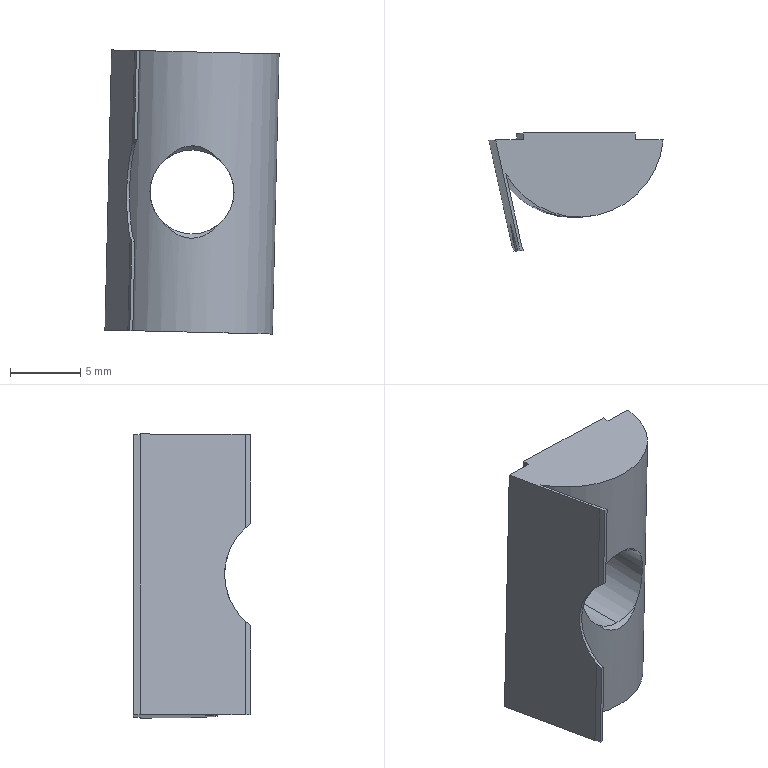Component | SolidWorks | 2012MB0201-1_UpperRackCoverModule-1_AHL21-308-M6-10 | 1 solid | 24 faces | box 12.43 x 8.39 x 20.28 mm | volume 945 mm3 | plane 11 | cylinder 8 | cone 5 | commonest cylinder face diameters 6 x2 11.084 x2 10.684 x2 12 x1 9 x1 | material S45C
STEP:
#1=CARTESIAN_POINT('',(-69.818,40.918,-25.855));
#2=VERTEX_POINT('',#1);
#3=CARTESIAN_POINT('',(-69.823,40.918,-26.091));
#4=VERTEX_POINT('',#3);
#5=CARTESIAN_POINT('',(-69.821,40.918,-25.973));
#6=DIRECTION('',(-0.,1.,0.));
#7=DIRECTION('',(-0.02392,0.,-0.9997));
#8=AXIS2_PLACEMENT_3D('',#5,#6,#7);
#9=CIRCLE('',#8,0.1181);
#10=EDGE_CURVE('',#2,#4,#9,.T.);
#11=ORIENTED_EDGE('',*,*,#10,.F.);
#12=CARTESIAN_POINT('',(-69.817,40.939,-25.834));
#13=VERTEX_POINT('',#12);
#14=CARTESIAN_POINT('',(-69.817,40.939,-25.834));
#15=DIRECTION('',(0.01691,0.7071,0.7069));
#16=VECTOR('',#15,39.37);
#17=LINE('',#14,#16);
#18=EDGE_CURVE('',#2,#13,#17,.T.);
#19=ORIENTED_EDGE('',*,*,#18,.T.);
#20=CARTESIAN_POINT('',(-69.824,40.939,-26.113));
#21=VERTEX_POINT('',#20);
#22=CARTESIAN_POINT('',(-69.821,40.939,-25.973));
#23=DIRECTION('',(0.,-1.,-0.));
#24=DIRECTION('',(0.9997,0.,-0.02392));
#25=AXIS2_PLACEMENT_3D('',#22,#23,#24);
#26=CIRCLE('',#25,0.1395);
#27=EDGE_CURVE('',#21,#13,#26,.T.);
#28=ORIENTED_EDGE('',*,*,#27,.F.);
#29=CARTESIAN_POINT('',(-69.824,40.939,-26.113));
#30=DIRECTION('',(-0.01691,0.7071,-0.7069));
#31=VECTOR('',#30,39.37);
#32=LINE('',#29,#31);
#33=EDGE_CURVE('',#4,#21,#32,.T.);
#34=ORIENTED_EDGE('',*,*,#33,.F.);
#35=EDGE_LOOP('',(#11,#19,#28,#34));
#36=FACE_OUTER_BOUND('',#35,.T.);
#37=CARTESIAN_POINT('',(-69.821,40.939,-25.973));
#38=DIRECTION('',(-0.,1.,0.));
#39=DIRECTION('',(-0.02392,0.,-0.9997));
#40=AXIS2_PLACEMENT_3D('',#37,#38,#39);
#41=CONICAL_SURFACE('',#40,0.1395,0.7854);
#42=ADVANCED_FACE('',(#36),#41,.F.);
#43=CARTESIAN_POINT('',(-69.818,40.715,-25.855));
#44=VERTEX_POINT('',#43);
#45=CARTESIAN_POINT('',(-69.892,40.715,-25.879));
#46=VERTEX_POINT('',#45);
#47=CARTESIAN_POINT('',(-69.821,40.715,-25.973));
#48=DIRECTION('',(0.,-1.,-0.));
#49=DIRECTION('',(0.02392,0.,0.9997));
#50=AXIS2_PLACEMENT_3D('',#47,#48,#49);
#51=CIRCLE('',#50,0.1181);
#52=EDGE_CURVE('',#44,#46,#51,.T.);
#53=ORIENTED_EDGE('',*,*,#52,.F.);
#54=CARTESIAN_POINT('',(-69.817,40.703,-25.843));
#55=VERTEX_POINT('',#54);
#56=CARTESIAN_POINT('',(-69.817,40.703,-25.843));
#57=DIRECTION('',(0.01691,-0.7071,0.7069));
#58=VECTOR('',#57,39.37);
#59=LINE('',#56,#58);
#60=EDGE_CURVE('',#44,#55,#59,.T.);
#61=ORIENTED_EDGE('',*,*,#60,.T.);
#62=CARTESIAN_POINT('',(-69.817,40.703,-25.843));
#63=CARTESIAN_POINT('',(-69.825,40.703,-25.843));
#64=CARTESIAN_POINT('',(-69.832,40.703,-25.844));
#65=CARTESIAN_POINT('',(-69.846,40.704,-25.847));
#66=CARTESIAN_POINT('',(-69.853,40.705,-25.85));
#67=CARTESIAN_POINT('',(-69.865,40.708,-25.856));
#68=CARTESIAN_POINT('',(-69.871,40.709,-25.86));
#69=CARTESIAN_POINT('',(-69.882,40.712,-25.869));
#70=CARTESIAN_POINT('',(-69.887,40.713,-25.874));
#71=CARTESIAN_POINT('',(-69.892,40.715,-25.879));
#72=B_SPLINE_CURVE_WITH_KNOTS('',3,(#62,#63,#64,#65,#66,#67,#68,#69,#70,#71),.UNSPECIFIED.,.F.,.F.,(4,2,2,2,4),(0.002342,0.002889,0.003436,0.003983,0.00453),.UNSPECIFIED.);
#73=EDGE_CURVE('',#55,#46,#72,.T.);
#74=ORIENTED_EDGE('',*,*,#73,.T.);
#75=EDGE_LOOP('',(#53,#61,#74));
#76=FACE_OUTER_BOUND('',#75,.T.);
#77=CARTESIAN_POINT('',(-69.821,40.703,-25.973));
#78=DIRECTION('',(0.,-1.,-0.));
#79=DIRECTION('',(0.02392,0.,0.9997));
#80=AXIS2_PLACEMENT_3D('',#77,#78,#79);
#81=CONICAL_SURFACE('',#80,0.1299,0.7854);
#82=ADVANCED_FACE('',(#76),#81,.F.);
#83=ORIENTED_EDGE('',*,*,#10,.T.);
#84=CARTESIAN_POINT('',(-69.823,40.715,-26.091));
#85=VERTEX_POINT('',#84);
#86=CARTESIAN_POINT('',(-69.823,40.703,-26.091));
#87=DIRECTION('',(0.,-1.,-0.));
#88=VECTOR('',#87,39.37);
#89=LINE('',#86,#88);
#90=EDGE_CURVE('',#4,#85,#89,.T.);
#91=ORIENTED_EDGE('',*,*,#90,.T.);
#92=CARTESIAN_POINT('',(-69.749,40.715,-26.067));
#93=VERTEX_POINT('',#92);
#94=CARTESIAN_POINT('',(-69.821,40.715,-25.973));
#95=DIRECTION('',(0.,-1.,-0.));
#96=DIRECTION('',(0.02392,0.,0.9997));
#97=AXIS2_PLACEMENT_3D('',#94,#95,#96);
#98=CIRCLE('',#97,0.1181);
#99=EDGE_CURVE('',#85,#93,#98,.T.);
#100=ORIENTED_EDGE('',*,*,#99,.T.);
#101=CARTESIAN_POINT('',(-69.745,40.715,-25.883));
#102=VERTEX_POINT('',#101);
#103=CARTESIAN_POINT('',(-69.749,40.715,-26.067));
#104=CARTESIAN_POINT('',(-69.742,40.717,-26.062));
#105=CARTESIAN_POINT('',(-69.736,40.719,-26.056));
#106=CARTESIAN_POINT('',(-69.725,40.724,-26.043));
#107=CARTESIAN_POINT('',(-69.72,40.726,-26.035));
#108=CARTESIAN_POINT('',(-69.712,40.73,-26.02));
#109=CARTESIAN_POINT('',(-69.708,40.731,-26.012));
#110=CARTESIAN_POINT('',(-69.704,40.734,-25.994));
#111=CARTESIAN_POINT('',(-69.703,40.734,-25.985));
#112=CARTESIAN_POINT('',(-69.702,40.734,-25.967));
#113=CARTESIAN_POINT('',(-69.703,40.734,-25.958));
#114=CARTESIAN_POINT('',(-69.707,40.732,-25.941));
#115=CARTESIAN_POINT('',(-69.709,40.73,-25.932));
#116=CARTESIAN_POINT('',(-69.717,40.726,-25.916));
#117=CARTESIAN_POINT('',(-69.721,40.724,-25.909));
#118=CARTESIAN_POINT('',(-69.732,40.719,-25.895));
#119=CARTESIAN_POINT('',(-69.738,40.717,-25.889));
#120=CARTESIAN_POINT('',(-69.745,40.715,-25.883));
#121=B_SPLINE_CURVE_WITH_KNOTS('',3,(#103,#104,#105,#106,#107,#108,#109,#110,#111,#112,#113,#114,#115,#116,#117,#118,#119,#120),.UNSPECIFIED.,.F.,.F.,(4,2,2,2,2,2,2,2,4),(0.,0.0006822,0.001364,0.002046,0.002729,0.003411,0.004093,0.004775,0.005457),.UNSPECIFIED.);
#122=EDGE_CURVE('',#93,#102,#121,.T.);
#123=ORIENTED_EDGE('',*,*,#122,.T.);
#124=CARTESIAN_POINT('',(-69.821,40.715,-25.973));
#125=DIRECTION('',(0.,-1.,-0.));
#126=DIRECTION('',(0.02392,0.,0.9997));
#127=AXIS2_PLACEMENT_3D('',#124,#125,#126);
#128=CIRCLE('',#127,0.1181);
#129=EDGE_CURVE('',#102,#44,#128,.T.);
#130=ORIENTED_EDGE('',*,*,#129,.T.);
#131=CARTESIAN_POINT('',(-69.818,40.703,-25.855));
#132=DIRECTION('',(0.,-1.,-0.));
#133=VECTOR('',#132,39.37);
#134=LINE('',#131,#133);
#135=EDGE_CURVE('',#2,#44,#134,.T.);
#136=ORIENTED_EDGE('',*,*,#135,.F.);
#137=EDGE_LOOP('',(#83,#91,#100,#123,#130,#136));
#138=FACE_OUTER_BOUND('',#137,.T.);
#139=CARTESIAN_POINT('',(-69.821,40.703,-25.973));
#140=DIRECTION('',(0.,-1.,-0.));
#141=DIRECTION('',(0.02392,0.,0.9997));
#142=AXIS2_PLACEMENT_3D('',#139,#140,#141);
#143=CYLINDRICAL_SURFACE('',#142,0.1181);
#144=ADVANCED_FACE('',(#138),#143,.F.);
#145=CARTESIAN_POINT('',(-69.99,40.609,-26.113));
#146=VERTEX_POINT('',#145);
#147=CARTESIAN_POINT('',(-69.995,40.609,-26.363));
#148=VERTEX_POINT('',#147);
#149=CARTESIAN_POINT('',(-69.977,40.609,-25.576));
#150=DIRECTION('',(-0.02392,0.,-0.9997));
#151=VECTOR('',#150,39.37);
#152=LINE('',#149,#151);
#153=EDGE_CURVE('',#146,#148,#152,.T.);
#154=ORIENTED_EDGE('',*,*,#153,.F.);
#155=CARTESIAN_POINT('',(-69.994,40.625,-26.1));
#156=VERTEX_POINT('',#155);
#157=CARTESIAN_POINT('',(-69.994,40.625,-26.1));
#158=CARTESIAN_POINT('',(-69.993,40.619,-26.105));
#159=CARTESIAN_POINT('',(-69.991,40.614,-26.109));
#160=CARTESIAN_POINT('',(-69.99,40.609,-26.113));
#161=B_SPLINE_CURVE_WITH_KNOTS('',3,(#157,#158,#159,#160),.UNSPECIFIED.,.F.,.F.,(4,4),(0.,0.0005334),.UNSPECIFIED.);
#162=EDGE_CURVE('',#156,#146,#161,.T.);
#163=ORIENTED_EDGE('',*,*,#162,.F.);
#164=CARTESIAN_POINT('',(-70.001,40.625,-26.363));
#165=VERTEX_POINT('',#164);
#166=CARTESIAN_POINT('',(-69.982,40.625,-25.576));
#167=DIRECTION('',(-0.02392,0.,-0.9997));
#168=VECTOR('',#167,39.37);
#169=LINE('',#166,#168);
#170=EDGE_CURVE('',#156,#165,#169,.T.);
#171=ORIENTED_EDGE('',*,*,#170,.T.);
#172=CARTESIAN_POINT('',(-69.791,40.685,-26.368));
#173=DIRECTION('',(-0.02392,0.,-0.9997));
#174=DIRECTION('',(-0.9997,0.,0.02392));
#175=AXIS2_PLACEMENT_3D('',#172,#173,#174);
#176=CIRCLE('',#175,0.2182);
#177=EDGE_CURVE('',#148,#165,#176,.T.);
#178=ORIENTED_EDGE('',*,*,#177,.F.);
#179=EDGE_LOOP('',(#154,#163,#171,#178));
#180=FACE_OUTER_BOUND('',#179,.T.);
#181=CARTESIAN_POINT('',(-69.772,40.685,-25.581));
#182=DIRECTION('',(-0.02392,0.,-0.9997));
#183=DIRECTION('',(-0.9997,0.,0.02392));
#184=AXIS2_PLACEMENT_3D('',#181,#182,#183);
#185=CYLINDRICAL_SURFACE('',#184,0.2182);
#186=ADVANCED_FACE('',(#180),#185,.T.);
#187=CARTESIAN_POINT('',(-69.974,40.609,-25.826));
#188=VERTEX_POINT('',#187);
#189=CARTESIAN_POINT('',(-69.968,40.609,-25.576));
#190=VERTEX_POINT('',#189);
#191=CARTESIAN_POINT('',(-69.968,40.609,-25.576));
#192=DIRECTION('',(0.02392,-0.,0.9997));
#193=VECTOR('',#192,39.37);
#194=LINE('',#191,#193);
#195=EDGE_CURVE('',#188,#190,#194,.T.);
#196=ORIENTED_EDGE('',*,*,#195,.F.);
#197=CARTESIAN_POINT('',(-69.981,40.626,-25.84));
#198=VERTEX_POINT('',#197);
#199=CARTESIAN_POINT('',(-69.981,40.626,-25.84));
#200=CARTESIAN_POINT('',(-69.979,40.621,-25.835));
#201=CARTESIAN_POINT('',(-69.977,40.615,-25.83));
#202=CARTESIAN_POINT('',(-69.974,40.609,-25.826));
#203=B_SPLINE_CURVE_WITH_KNOTS('',3,(#199,#200,#201,#202),.UNSPECIFIED.,.F.,.F.,(4,4),(0.,0.0006031),.UNSPECIFIED.);
#204=EDGE_CURVE('',#198,#188,#203,.T.);
#205=ORIENTED_EDGE('',*,*,#204,.F.);
#206=CARTESIAN_POINT('',(-69.974,40.626,-25.576));
#207=VERTEX_POINT('',#206);
#208=CARTESIAN_POINT('',(-69.974,40.626,-25.576));
#209=DIRECTION('',(-0.02392,0.,-0.9997));
#210=VECTOR('',#209,39.37);
#211=LINE('',#208,#210);
#212=EDGE_CURVE('',#207,#198,#211,.T.);
#213=ORIENTED_EDGE('',*,*,#212,.F.);
#214=CARTESIAN_POINT('',(-69.772,40.685,-25.581));
#215=DIRECTION('',(0.02392,-0.,0.9997));
#216=DIRECTION('',(0.9997,0.,-0.02392));
#217=AXIS2_PLACEMENT_3D('',#214,#215,#216);
#218=CIRCLE('',#217,0.2103);
#219=EDGE_CURVE('',#207,#190,#218,.T.);
#220=ORIENTED_EDGE('',*,*,#219,.T.);
#221=EDGE_LOOP('',(#196,#205,#213,#220));
#222=FACE_OUTER_BOUND('',#221,.T.);
#223=CARTESIAN_POINT('',(-69.772,40.685,-25.581));
#224=DIRECTION('',(-0.02392,0.,-0.9997));
#225=DIRECTION('',(-0.9997,0.,0.02392));
#226=AXIS2_PLACEMENT_3D('',#223,#224,#225);
#227=CYLINDRICAL_SURFACE('',#226,0.2103);
#228=ADVANCED_FACE('',(#222),#227,.F.);
#229=CARTESIAN_POINT('',(-69.987,40.919,-26.363));
#230=VERTEX_POINT('',#229);
#231=CARTESIAN_POINT('',(-69.987,40.939,-26.363));
#232=VERTEX_POINT('',#231);
#233=CARTESIAN_POINT('',(-69.987,40.919,-26.363));
#234=DIRECTION('',(-0.,1.,0.));
#235=VECTOR('',#234,39.37);
#236=LINE('',#233,#235);
#237=EDGE_CURVE('',#230,#232,#236,.T.);
#238=ORIENTED_EDGE('',*,*,#237,.F.);
#239=CARTESIAN_POINT('',(-69.969,40.919,-25.576));
#240=VERTEX_POINT('',#239);
#241=CARTESIAN_POINT('',(-69.969,40.919,-25.576));
#242=DIRECTION('',(-0.02392,0.,-0.9997));
#243=VECTOR('',#242,39.37);
#244=LINE('',#241,#243);
#245=EDGE_CURVE('',#240,#230,#244,.T.);
#246=ORIENTED_EDGE('',*,*,#245,.F.);
#247=CARTESIAN_POINT('',(-69.969,40.939,-25.576));
#248=VERTEX_POINT('',#247);
#249=CARTESIAN_POINT('',(-69.969,40.919,-25.576));
#250=DIRECTION('',(-0.,1.,0.));
#251=VECTOR('',#250,39.37);
#252=LINE('',#249,#251);
#253=EDGE_CURVE('',#240,#248,#252,.T.);
#254=ORIENTED_EDGE('',*,*,#253,.T.);
#255=CARTESIAN_POINT('',(-69.969,40.939,-25.576));
#256=DIRECTION('',(-0.02392,0.,-0.9997));
#257=VECTOR('',#256,39.37);
#258=LINE('',#255,#257);
#259=EDGE_CURVE('',#248,#232,#258,.T.);
#260=ORIENTED_EDGE('',*,*,#259,.T.);
#261=EDGE_LOOP('',(#238,#246,#254,#260));
#262=FACE_OUTER_BOUND('',#261,.T.);
#263=CARTESIAN_POINT('',(-69.969,40.919,-25.576));
#264=DIRECTION('',(-0.9997,-0.,0.02392));
#265=DIRECTION('',(0.02392,-0.,0.9997));
#266=AXIS2_PLACEMENT_3D('',#263,#264,#265);
#267=PLANE('',#266);
#268=ADVANCED_FACE('',(#262),#267,.T.);
#269=CARTESIAN_POINT('',(-70.065,40.919,-26.361));
#270=VERTEX_POINT('',#269);
#271=CARTESIAN_POINT('',(-70.065,40.919,-26.361));
#272=DIRECTION('',(0.9997,0.,-0.02392));
#273=VECTOR('',#272,39.37);
#274=LINE('',#271,#273);
#275=EDGE_CURVE('',#270,#230,#274,.T.);
#276=ORIENTED_EDGE('',*,*,#275,.F.);
#277=CARTESIAN_POINT('',(-70.046,40.919,-25.574));
#278=VERTEX_POINT('',#277);
#279=CARTESIAN_POINT('',(-70.046,40.919,-25.574));
#280=DIRECTION('',(-0.02392,0.,-0.9997));
#281=VECTOR('',#280,39.37);
#282=LINE('',#279,#281);
#283=EDGE_CURVE('',#278,#270,#282,.T.);
#284=ORIENTED_EDGE('',*,*,#283,.F.);
#285=CARTESIAN_POINT('',(-70.046,40.919,-25.574));
#286=DIRECTION('',(0.9997,0.,-0.02392));
#287=VECTOR('',#286,39.37);
#288=LINE('',#285,#287);
#289=EDGE_CURVE('',#278,#240,#288,.T.);
#290=ORIENTED_EDGE('',*,*,#289,.T.);
#291=ORIENTED_EDGE('',*,*,#245,.T.);
#292=EDGE_LOOP('',(#276,#284,#290,#291));
#293=FACE_OUTER_BOUND('',#292,.T.);
#294=CARTESIAN_POINT('',(-70.046,40.919,-25.574));
#295=DIRECTION('',(-0.,1.,0.));
#296=DIRECTION('',(0.9997,0.,-0.02392));
#297=AXIS2_PLACEMENT_3D('',#294,#295,#296);
#298=PLANE('',#297);
#299=ADVANCED_FACE('',(#293),#298,.T.);
#300=ORIENTED_EDGE('',*,*,#170,.F.);
#301=CARTESIAN_POINT('',(-69.988,40.625,-25.838));
#302=VERTEX_POINT('',#301);
#303=CARTESIAN_POINT('',(-69.988,40.625,-25.838));
#304=CARTESIAN_POINT('',(-70.008,40.707,-25.913));
#305=CARTESIAN_POINT('',(-70.011,40.707,-26.025));
#306=CARTESIAN_POINT('',(-69.994,40.625,-26.1));
#307=(BOUNDED_CURVE()B_SPLINE_CURVE(3,(#303,#304,#305,#306),.UNSPECIFIED.,.F.,.F.)B_SPLINE_CURVE_WITH_KNOTS((4,4),(5.451,7.115),.UNSPECIFIED.)CURVE()GEOMETRIC_REPRESENTATION_ITEM()RATIONAL_B_SPLINE_CURVE((1.,0.7821,0.7821,1.))REPRESENTATION_ITEM(''));
#308=EDGE_CURVE('',#302,#156,#307,.T.);
#309=ORIENTED_EDGE('',*,*,#308,.F.);
#310=CARTESIAN_POINT('',(-69.982,40.625,-25.576));
#311=VERTEX_POINT('',#310);
#312=CARTESIAN_POINT('',(-69.982,40.625,-25.576));
#313=DIRECTION('',(-0.02392,0.,-0.9997));
#314=VECTOR('',#313,39.37);
#315=LINE('',#312,#314);
#316=EDGE_CURVE('',#311,#302,#315,.T.);
#317=ORIENTED_EDGE('',*,*,#316,.F.);
#318=CARTESIAN_POINT('',(-69.982,40.625,-25.576));
#319=DIRECTION('',(-0.214,0.9768,0.005122));
#320=VECTOR('',#319,39.37);
#321=LINE('',#318,#320);
#322=EDGE_CURVE('',#311,#278,#321,.T.);
#323=ORIENTED_EDGE('',*,*,#322,.T.);
#324=ORIENTED_EDGE('',*,*,#283,.T.);
#325=CARTESIAN_POINT('',(-70.001,40.625,-26.363));
#326=DIRECTION('',(-0.214,0.9768,0.005122));
#327=VECTOR('',#326,39.37);
#328=LINE('',#325,#327);
#329=EDGE_CURVE('',#165,#270,#328,.T.);
#330=ORIENTED_EDGE('',*,*,#329,.F.);
#331=EDGE_LOOP('',(#300,#309,#317,#323,#324,#330));
#332=FACE_OUTER_BOUND('',#331,.T.);
#333=CARTESIAN_POINT('',(-69.982,40.625,-25.576));
#334=DIRECTION('',(-0.9765,-0.2141,0.02337));
#335=DIRECTION('',(-0.214,0.9768,0.005122));
#336=AXIS2_PLACEMENT_3D('',#333,#334,#335);
#337=PLANE('',#336);
#338=ADVANCED_FACE('',(#332),#337,.T.);
#339=CARTESIAN_POINT('',(-69.977,40.609,-25.576));
#340=VERTEX_POINT('',#339);
#341=CARTESIAN_POINT('',(-69.983,40.609,-25.826));
#342=VERTEX_POINT('',#341);
#343=CARTESIAN_POINT('',(-69.977,40.609,-25.576));
#344=DIRECTION('',(-0.02392,0.,-0.9997));
#345=VECTOR('',#344,39.37);
#346=LINE('',#343,#345);
#347=EDGE_CURVE('',#340,#342,#346,.T.);
#348=ORIENTED_EDGE('',*,*,#347,.F.);
#349=CARTESIAN_POINT('',(-69.772,40.685,-25.581));
#350=DIRECTION('',(-0.02392,0.,-0.9997));
#351=DIRECTION('',(-0.9997,0.,0.02392));
#352=AXIS2_PLACEMENT_3D('',#349,#350,#351);
#353=CIRCLE('',#352,0.2182);
#354=EDGE_CURVE('',#340,#311,#353,.T.);
#355=ORIENTED_EDGE('',*,*,#354,.T.);
#356=ORIENTED_EDGE('',*,*,#316,.T.);
#357=CARTESIAN_POINT('',(-69.983,40.609,-25.826));
#358=CARTESIAN_POINT('',(-69.985,40.614,-25.829));
#359=CARTESIAN_POINT('',(-69.987,40.619,-25.834));
#360=CARTESIAN_POINT('',(-69.988,40.625,-25.838));
#361=B_SPLINE_CURVE_WITH_KNOTS('',3,(#357,#358,#359,#360),.UNSPECIFIED.,.F.,.F.,(4,4),(0.005895,0.006427),.UNSPECIFIED.);
#362=EDGE_CURVE('',#342,#302,#361,.T.);
#363=ORIENTED_EDGE('',*,*,#362,.F.);
#364=EDGE_LOOP('',(#348,#355,#356,#363));
#365=FACE_OUTER_BOUND('',#364,.T.);
#366=CARTESIAN_POINT('',(-69.772,40.685,-25.581));
#367=DIRECTION('',(-0.02392,0.,-0.9997));
#368=DIRECTION('',(-0.9997,0.,0.02392));
#369=AXIS2_PLACEMENT_3D('',#366,#367,#368);
#370=CYLINDRICAL_SURFACE('',#369,0.2182);
#371=ADVANCED_FACE('',(#365),#370,.T.);
#372=CARTESIAN_POINT('',(-69.987,40.609,-26.363));
#373=VERTEX_POINT('',#372);
#374=CARTESIAN_POINT('',(-69.981,40.609,-26.113));
#375=VERTEX_POINT('',#374);
#376=CARTESIAN_POINT('',(-69.968,40.609,-25.576));
#377=DIRECTION('',(0.02392,-0.,0.9997));
#378=VECTOR('',#377,39.37);
#379=LINE('',#376,#378);
#380=EDGE_CURVE('',#373,#375,#379,.T.);
#381=ORIENTED_EDGE('',*,*,#380,.F.);
#382=CARTESIAN_POINT('',(-69.993,40.626,-26.363));
#383=VERTEX_POINT('',#382);
#384=CARTESIAN_POINT('',(-69.791,40.685,-26.368));
#385=DIRECTION('',(0.02392,-0.,0.9997));
#386=DIRECTION('',(0.9997,0.,-0.02392));
#387=AXIS2_PLACEMENT_3D('',#384,#385,#386);
#388=CIRCLE('',#387,0.2103);
#389=EDGE_CURVE('',#383,#373,#388,.T.);
#390=ORIENTED_EDGE('',*,*,#389,.F.);
#391=CARTESIAN_POINT('',(-69.987,40.626,-26.099));
#392=VERTEX_POINT('',#391);
#393=CARTESIAN_POINT('',(-69.974,40.626,-25.576));
#394=DIRECTION('',(-0.02392,0.,-0.9997));
#395=VECTOR('',#394,39.37);
#396=LINE('',#393,#395);
#397=EDGE_CURVE('',#392,#383,#396,.T.);
#398=ORIENTED_EDGE('',*,*,#397,.F.);
#399=CARTESIAN_POINT('',(-69.981,40.609,-26.113));
#400=CARTESIAN_POINT('',(-69.983,40.615,-26.109));
#401=CARTESIAN_POINT('',(-69.985,40.621,-26.104));
#402=CARTESIAN_POINT('',(-69.987,40.626,-26.099));
#403=B_SPLINE_CURVE_WITH_KNOTS('',3,(#399,#400,#401,#402),.UNSPECIFIED.,.F.,.F.,(4,4),(0.005576,0.006177),.UNSPECIFIED.);
#404=EDGE_CURVE('',#375,#392,#403,.T.);
#405=ORIENTED_EDGE('',*,*,#404,.F.);
#406=EDGE_LOOP('',(#381,#390,#398,#405));
#407=FACE_OUTER_BOUND('',#406,.T.);
#408=CARTESIAN_POINT('',(-69.772,40.685,-25.581));
#409=DIRECTION('',(-0.02392,0.,-0.9997));
#410=DIRECTION('',(-0.9997,0.,0.02392));
#411=AXIS2_PLACEMENT_3D('',#408,#409,#410);
#412=CYLINDRICAL_SURFACE('',#411,0.2103);
#413=ADVANCED_FACE('',(#407),#412,.F.);
#414=CARTESIAN_POINT('',(-69.987,40.626,-26.099));
#415=CARTESIAN_POINT('',(-70.002,40.706,-26.024));
#416=CARTESIAN_POINT('',(-70.,40.706,-25.914));
#417=CARTESIAN_POINT('',(-69.981,40.626,-25.84));
#418=(BOUNDED_CURVE()B_SPLINE_CURVE(3,(#414,#415,#416,#417),.UNSPECIFIED.,.F.,.F.)B_SPLINE_CURVE_WITH_KNOTS((4,4),(5.466,7.101),.UNSPECIFIED.)CURVE()GEOMETRIC_REPRESENTATION_ITEM()RATIONAL_B_SPLINE_CURVE((1.,0.7894,0.7894,1.))REPRESENTATION_ITEM(''));
#419=EDGE_CURVE('',#392,#198,#418,.T.);
#420=ORIENTED_EDGE('',*,*,#419,.F.);
#421=ORIENTED_EDGE('',*,*,#397,.T.);
#422=CARTESIAN_POINT('',(-70.036,40.824,-26.362));
#423=VERTEX_POINT('',#422);
#424=CARTESIAN_POINT('',(-70.036,40.824,-26.362));
#425=DIRECTION('',(0.2142,-0.9768,-0.005124));
#426=VECTOR('',#425,39.37);
#427=LINE('',#424,#426);
#428=EDGE_CURVE('',#423,#383,#427,.T.);
#429=ORIENTED_EDGE('',*,*,#428,.F.);
#430=CARTESIAN_POINT('',(-70.018,40.824,-25.575));
#431=VERTEX_POINT('',#430);
#432=CARTESIAN_POINT('',(-70.018,40.824,-25.575));
#433=DIRECTION('',(-0.02392,0.,-0.9997));
#434=VECTOR('',#433,39.37);
#435=LINE('',#432,#434);
#436=EDGE_CURVE('',#431,#423,#435,.T.);
#437=ORIENTED_EDGE('',*,*,#436,.F.);
#438=CARTESIAN_POINT('',(-70.018,40.824,-25.575));
#439=DIRECTION('',(0.2142,-0.9768,-0.005124));
#440=VECTOR('',#439,39.37);
#441=LINE('',#438,#440);
#442=EDGE_CURVE('',#431,#207,#441,.T.);
#443=ORIENTED_EDGE('',*,*,#442,.T.);
#444=ORIENTED_EDGE('',*,*,#212,.T.);
#445=EDGE_LOOP('',(#420,#421,#429,#437,#443,#444));
#446=FACE_OUTER_BOUND('',#445,.T.);
#447=CARTESIAN_POINT('',(-70.018,40.824,-25.575));
#448=DIRECTION('',(0.9765,0.2142,-0.02337));
#449=DIRECTION('',(0.2142,-0.9768,-0.005124));
#450=AXIS2_PLACEMENT_3D('',#447,#448,#449);
#451=PLANE('',#450);
#452=ADVANCED_FACE('',(#446),#451,.T.);
#453=CARTESIAN_POINT('',(-69.896,40.715,-26.064));
#454=VERTEX_POINT('',#453);
#455=CARTESIAN_POINT('',(-69.896,40.715,-26.064));
#456=CARTESIAN_POINT('',(-69.892,40.713,-26.069));
#457=CARTESIAN_POINT('',(-69.887,40.712,-26.075));
#458=CARTESIAN_POINT('',(-69.877,40.709,-26.084));
#459=CARTESIAN_POINT('',(-69.871,40.708,-26.088));
#460=CARTESIAN_POINT('',(-69.859,40.705,-26.095));
#461=CARTESIAN_POINT('',(-69.852,40.704,-26.098));
#462=CARTESIAN_POINT('',(-69.838,40.703,-26.102));
#463=CARTESIAN_POINT('',(-69.831,40.703,-26.103));
#464=CARTESIAN_POINT('',(-69.817,40.703,-26.103));
#465=CARTESIAN_POINT('',(-69.809,40.703,-26.103));
#466=CARTESIAN_POINT('',(-69.795,40.704,-26.099));
#467=CARTESIAN_POINT('',(-69.788,40.705,-26.097));
#468=CARTESIAN_POINT('',(-69.776,40.707,-26.09));
#469=CARTESIAN_POINT('',(-69.77,40.709,-26.087));
#470=CARTESIAN_POINT('',(-69.759,40.712,-26.078));
#471=CARTESIAN_POINT('',(-69.754,40.713,-26.073));
#472=CARTESIAN_POINT('',(-69.749,40.715,-26.067));
#473=B_SPLINE_CURVE_WITH_KNOTS('',3,(#455,#456,#457,#458,#459,#460,#461,#462,#463,#464,#465,#466,#467,#468,#469,#470,#471,#472),.UNSPECIFIED.,.F.,.F.,(4,2,2,2,2,2,2,2,4),(0.0001474,0.0006953,0.001243,0.001791,0.002339,0.002887,0.003435,0.003983,0.00453),.UNSPECIFIED.);
#474=EDGE_CURVE('',#454,#93,#473,.T.);
#475=ORIENTED_EDGE('',*,*,#474,.F.);
#476=CARTESIAN_POINT('',(-69.892,40.715,-25.879));
#477=CARTESIAN_POINT('',(-69.899,40.717,-25.885));
#478=CARTESIAN_POINT('',(-69.905,40.719,-25.891));
#479=CARTESIAN_POINT('',(-69.916,40.724,-25.904));
#480=CARTESIAN_POINT('',(-69.921,40.726,-25.911));
#481=CARTESIAN_POINT('',(-69.929,40.73,-25.927));
#482=CARTESIAN_POINT('',(-69.933,40.731,-25.935));
#483=CARTESIAN_POINT('',(-69.937,40.734,-25.952));
#484=CARTESIAN_POINT('',(-69.938,40.734,-25.961));
#485=CARTESIAN_POINT('',(-69.939,40.734,-25.979));
#486=CARTESIAN_POINT('',(-69.938,40.734,-25.988));
#487=CARTESIAN_POINT('',(-69.934,40.732,-26.006));
#488=CARTESIAN_POINT('',(-69.932,40.73,-26.014));
#489=CARTESIAN_POINT('',(-69.924,40.726,-26.03));
#490=CARTESIAN_POINT('',(-69.92,40.724,-26.038));
#491=CARTESIAN_POINT('',(-69.909,40.719,-26.052));
#492=CARTESIAN_POINT('',(-69.903,40.717,-26.058));
#493=CARTESIAN_POINT('',(-69.896,40.715,-26.064));
#494=B_SPLINE_CURVE_WITH_KNOTS('',3,(#476,#477,#478,#479,#480,#481,#482,#483,#484,#485,#486,#487,#488,#489,#490,#491,#492,#493),.UNSPECIFIED.,.F.,.F.,(4,2,2,2,2,2,2,2,4),(0.,0.0006822,0.001364,0.002046,0.002729,0.003411,0.004093,0.004775,0.005457),.UNSPECIFIED.);
#495=EDGE_CURVE('',#46,#454,#494,.T.);
#496=ORIENTED_EDGE('',*,*,#495,.F.);
#497=ORIENTED_EDGE('',*,*,#73,.F.);
#498=CARTESIAN_POINT('',(-69.745,40.715,-25.883));
#499=CARTESIAN_POINT('',(-69.749,40.713,-25.877));
#500=CARTESIAN_POINT('',(-69.754,40.712,-25.872));
#501=CARTESIAN_POINT('',(-69.764,40.709,-25.863));
#502=CARTESIAN_POINT('',(-69.77,40.707,-25.859));
#503=CARTESIAN_POINT('',(-69.783,40.705,-25.852));
#504=CARTESIAN_POINT('',(-69.789,40.704,-25.849));
#505=CARTESIAN_POINT('',(-69.803,40.703,-25.845));
#506=CARTESIAN_POINT('',(-69.81,40.703,-25.844));
#507=CARTESIAN_POINT('',(-69.817,40.703,-25.843));
#508=B_SPLINE_CURVE_WITH_KNOTS('',3,(#498,#499,#500,#501,#502,#503,#504,#505,#506,#507),.UNSPECIFIED.,.F.,.F.,(4,2,2,2,4),(0.0001474,0.0006961,0.001245,0.001794,0.002342),.UNSPECIFIED.);
#509=EDGE_CURVE('',#102,#55,#508,.T.);
#510=ORIENTED_EDGE('',*,*,#509,.F.);
#511=ORIENTED_EDGE('',*,*,#122,.F.);
#512=EDGE_LOOP('',(#475,#496,#497,#510,#511));
#513=FACE_BOUND('',#512,.T.);
#514=CARTESIAN_POINT('',(-69.576,40.919,-25.585));
#515=VERTEX_POINT('',#514);
#516=CARTESIAN_POINT('',(-69.595,40.919,-26.373));
#517=VERTEX_POINT('',#516);
#518=CARTESIAN_POINT('',(-69.576,40.919,-25.585));
#519=DIRECTION('',(-0.02392,0.,-0.9997));
#520=VECTOR('',#519,39.37);
#521=LINE('',#518,#520);
#522=EDGE_CURVE('',#515,#517,#521,.T.);
#523=ORIENTED_EDGE('',*,*,#522,.F.);
#524=CARTESIAN_POINT('',(-69.811,40.939,-25.58));
#525=DIRECTION('',(-0.02392,0.,-0.9997));
#526=DIRECTION('',(-0.9997,0.,0.02392));
#527=AXIS2_PLACEMENT_3D('',#524,#525,#526);
#528=CIRCLE('',#527,0.2362);
#529=EDGE_CURVE('',#515,#431,#528,.T.);
#530=ORIENTED_EDGE('',*,*,#529,.T.);
#531=ORIENTED_EDGE('',*,*,#436,.T.);
#532=CARTESIAN_POINT('',(-69.83,40.939,-26.367));
#533=DIRECTION('',(-0.02392,0.,-0.9997));
#534=DIRECTION('',(-0.9997,0.,0.02392));
#535=AXIS2_PLACEMENT_3D('',#532,#533,#534);
#536=CIRCLE('',#535,0.2362);
#537=EDGE_CURVE('',#517,#423,#536,.T.);
#538=ORIENTED_EDGE('',*,*,#537,.F.);
#539=EDGE_LOOP('',(#523,#530,#531,#538));
#540=FACE_OUTER_BOUND('',#539,.T.);
#541=CARTESIAN_POINT('',(-69.811,40.939,-25.58));
#542=DIRECTION('',(-0.02392,0.,-0.9997));
#543=DIRECTION('',(-0.9997,0.,0.02392));
#544=AXIS2_PLACEMENT_3D('',#541,#542,#543);
#545=CYLINDRICAL_SURFACE('',#544,0.2362);
#546=ADVANCED_FACE('',(#513,#540),#545,.T.);
#547=ORIENTED_EDGE('',*,*,#27,.T.);
#548=CARTESIAN_POINT('',(-69.821,40.939,-25.973));
#549=DIRECTION('',(0.,-1.,-0.));
#550=DIRECTION('',(0.9997,0.,-0.02392));
#551=AXIS2_PLACEMENT_3D('',#548,#549,#550);
#552=CIRCLE('',#551,0.1395);
#553=EDGE_CURVE('',#13,#21,#552,.T.);
#554=ORIENTED_EDGE('',*,*,#553,.T.);
#555=EDGE_LOOP('',(#547,#554));
#556=FACE_BOUND('',#555,.T.);
#557=CARTESIAN_POINT('',(-69.654,40.939,-25.584));
#558=VERTEX_POINT('',#557);
#559=CARTESIAN_POINT('',(-69.673,40.939,-26.371));
#560=VERTEX_POINT('',#559);
#561=CARTESIAN_POINT('',(-69.654,40.939,-25.584));
#562=DIRECTION('',(-0.02392,0.,-0.9997));
#563=VECTOR('',#562,39.37);
#564=LINE('',#561,#563);
#565=EDGE_CURVE('',#558,#560,#564,.T.);
#566=ORIENTED_EDGE('',*,*,#565,.T.);
#567=CARTESIAN_POINT('',(-69.987,40.939,-26.363));
#568=DIRECTION('',(0.9997,0.,-0.02392));
#569=VECTOR('',#568,39.37);
#570=LINE('',#567,#569);
#571=EDGE_CURVE('',#232,#560,#570,.T.);
#572=ORIENTED_EDGE('',*,*,#571,.F.);
#573=ORIENTED_EDGE('',*,*,#259,.F.);
#574=CARTESIAN_POINT('',(-69.969,40.939,-25.576));
#575=DIRECTION('',(0.9997,0.,-0.02392));
#576=VECTOR('',#575,39.37);
#577=LINE('',#574,#576);
#578=EDGE_CURVE('',#248,#558,#577,.T.);
#579=ORIENTED_EDGE('',*,*,#578,.T.);
#580=EDGE_LOOP('',(#566,#572,#573,#579));
#581=FACE_OUTER_BOUND('',#580,.T.);
#582=CARTESIAN_POINT('',(-69.969,40.939,-25.576));
#583=DIRECTION('',(-0.,1.,0.));
#584=DIRECTION('',(0.9997,0.,-0.02392));
#585=AXIS2_PLACEMENT_3D('',#582,#583,#584);
#586=PLANE('',#585);
#587=ADVANCED_FACE('',(#556,#581),#586,.T.);
#588=ORIENTED_EDGE('',*,*,#354,.F.);
#589=CARTESIAN_POINT('',(-69.457,40.609,-25.588));
#590=DIRECTION('',(0.9997,0.,-0.02392));
#591=VECTOR('',#590,39.37);
#592=LINE('',#589,#591);
#593=EDGE_CURVE('',#340,#190,#592,.T.);
#594=ORIENTED_EDGE('',*,*,#593,.T.);
#595=ORIENTED_EDGE('',*,*,#219,.F.);
#596=ORIENTED_EDGE('',*,*,#442,.F.);
#597=ORIENTED_EDGE('',*,*,#529,.F.);
#598=CARTESIAN_POINT('',(-69.654,40.919,-25.584));
#599=VERTEX_POINT('',#598);
#600=CARTESIAN_POINT('',(-69.576,40.919,-25.585));
#601=DIRECTION('',(-0.9997,-0.,0.02392));
#602=VECTOR('',#601,39.37);
#603=LINE('',#600,#602);
#604=EDGE_CURVE('',#515,#599,#603,.T.);
#605=ORIENTED_EDGE('',*,*,#604,.T.);
#606=CARTESIAN_POINT('',(-69.654,40.919,-25.584));
#607=DIRECTION('',(-0.,1.,0.));
#608=VECTOR('',#607,39.37);
#609=LINE('',#606,#608);
#610=EDGE_CURVE('',#599,#558,#609,.T.);
#611=ORIENTED_EDGE('',*,*,#610,.T.);
#612=ORIENTED_EDGE('',*,*,#578,.F.);
#613=ORIENTED_EDGE('',*,*,#253,.F.);
#614=ORIENTED_EDGE('',*,*,#289,.F.);
#615=ORIENTED_EDGE('',*,*,#322,.F.);
#616=EDGE_LOOP('',(#588,#594,#595,#596,#597,#605,#611,#612,#613,#614,#615));
#617=FACE_OUTER_BOUND('',#616,.T.);
#618=CARTESIAN_POINT('',(-69.811,40.939,-25.58));
#619=DIRECTION('',(-0.02392,0.,-0.9997));
#620=DIRECTION('',(-0.9997,-0.,0.02392));
#621=AXIS2_PLACEMENT_3D('',#618,#619,#620);
#622=PLANE('',#621);
#623=ADVANCED_FACE('',(#617),#622,.F.);
#624=CARTESIAN_POINT('',(-69.83,40.609,-26.367));
#625=DIRECTION('',(0.9997,0.,-0.02392));
#626=VECTOR('',#625,39.37);
#627=LINE('',#624,#626);
#628=EDGE_CURVE('',#148,#373,#627,.T.);
#629=ORIENTED_EDGE('',*,*,#628,.F.);
#630=ORIENTED_EDGE('',*,*,#177,.T.);
#631=ORIENTED_EDGE('',*,*,#329,.T.);
#632=ORIENTED_EDGE('',*,*,#275,.T.);
#633=ORIENTED_EDGE('',*,*,#237,.T.);
#634=ORIENTED_EDGE('',*,*,#571,.T.);
#635=CARTESIAN_POINT('',(-69.673,40.919,-26.371));
#636=VERTEX_POINT('',#635);
#637=CARTESIAN_POINT('',(-69.673,40.919,-26.371));
#638=DIRECTION('',(-0.,1.,0.));
#639=VECTOR('',#638,39.37);
#640=LINE('',#637,#639);
#641=EDGE_CURVE('',#636,#560,#640,.T.);
#642=ORIENTED_EDGE('',*,*,#641,.F.);
#643=CARTESIAN_POINT('',(-69.595,40.919,-26.373));
#644=DIRECTION('',(-0.9997,-0.,0.02392));
#645=VECTOR('',#644,39.37);
#646=LINE('',#643,#645);
#647=EDGE_CURVE('',#517,#636,#646,.T.);
#648=ORIENTED_EDGE('',*,*,#647,.F.);
#649=ORIENTED_EDGE('',*,*,#537,.T.);
#650=ORIENTED_EDGE('',*,*,#428,.T.);
#651=ORIENTED_EDGE('',*,*,#389,.T.);
#652=EDGE_LOOP('',(#629,#630,#631,#632,#633,#634,#642,#648,#649,#650,#651));
#653=FACE_OUTER_BOUND('',#652,.T.);
#654=CARTESIAN_POINT('',(-69.83,40.939,-26.367));
#655=DIRECTION('',(-0.02392,0.,-0.9997));
#656=DIRECTION('',(-0.9997,-0.,0.02392));
#657=AXIS2_PLACEMENT_3D('',#654,#655,#656);
#658=PLANE('',#657);
#659=ADVANCED_FACE('',(#653),#658,.T.);
#660=ORIENTED_EDGE('',*,*,#647,.T.);
#661=CARTESIAN_POINT('',(-69.654,40.919,-25.584));
#662=DIRECTION('',(-0.02392,0.,-0.9997));
#663=VECTOR('',#662,39.37);
#664=LINE('',#661,#663);
#665=EDGE_CURVE('',#599,#636,#664,.T.);
#666=ORIENTED_EDGE('',*,*,#665,.F.);
#667=ORIENTED_EDGE('',*,*,#604,.F.);
#668=ORIENTED_EDGE('',*,*,#522,.T.);
#669=EDGE_LOOP('',(#660,#666,#667,#668));
#670=FACE_OUTER_BOUND('',#669,.T.);
#671=CARTESIAN_POINT('',(-69.576,40.919,-25.585));
#672=DIRECTION('',(0.,-1.,-0.));
#673=DIRECTION('',(0.02392,-0.,0.9997));
#674=AXIS2_PLACEMENT_3D('',#671,#672,#673);
#675=PLANE('',#674);
#676=ADVANCED_FACE('',(#670),#675,.F.);
#677=ORIENTED_EDGE('',*,*,#641,.T.);
#678=ORIENTED_EDGE('',*,*,#565,.F.);
#679=ORIENTED_EDGE('',*,*,#610,.F.);
#680=ORIENTED_EDGE('',*,*,#665,.T.);
#681=EDGE_LOOP('',(#677,#678,#679,#680));
#682=FACE_OUTER_BOUND('',#681,.T.);
#683=CARTESIAN_POINT('',(-69.654,40.919,-25.584));
#684=DIRECTION('',(-0.9997,-0.,0.02392));
#685=DIRECTION('',(0.02392,-0.,0.9997));
#686=AXIS2_PLACEMENT_3D('',#683,#684,#685);
#687=PLANE('',#686);
#688=ADVANCED_FACE('',(#682),#687,.F.);
#689=CARTESIAN_POINT('',(-69.821,40.715,-25.973));
#690=DIRECTION('',(0.,-1.,-0.));
#691=DIRECTION('',(0.02392,0.,0.9997));
#692=AXIS2_PLACEMENT_3D('',#689,#690,#691);
#693=CIRCLE('',#692,0.1181);
#694=EDGE_CURVE('',#454,#85,#693,.T.);
#695=ORIENTED_EDGE('',*,*,#694,.F.);
#696=ORIENTED_EDGE('',*,*,#474,.T.);
#697=ORIENTED_EDGE('',*,*,#99,.F.);
#698=EDGE_LOOP('',(#695,#696,#697));
#699=FACE_OUTER_BOUND('',#698,.T.);
#700=CARTESIAN_POINT('',(-69.821,40.703,-25.973));
#701=DIRECTION('',(0.,-1.,-0.));
#702=DIRECTION('',(0.02392,0.,0.9997));
#703=AXIS2_PLACEMENT_3D('',#700,#701,#702);
#704=CONICAL_SURFACE('',#703,0.1299,0.7854);
#705=ADVANCED_FACE('',(#699),#704,.F.);
#706=ORIENTED_EDGE('',*,*,#90,.F.);
#707=CARTESIAN_POINT('',(-69.821,40.918,-25.973));
#708=DIRECTION('',(-0.,1.,0.));
#709=DIRECTION('',(-0.02392,0.,-0.9997));
#710=AXIS2_PLACEMENT_3D('',#707,#708,#709);
#711=CIRCLE('',#710,0.1181);
#712=EDGE_CURVE('',#4,#2,#711,.T.);
#713=ORIENTED_EDGE('',*,*,#712,.T.);
#714=ORIENTED_EDGE('',*,*,#135,.T.);
#715=ORIENTED_EDGE('',*,*,#52,.T.);
#716=ORIENTED_EDGE('',*,*,#495,.T.);
#717=ORIENTED_EDGE('',*,*,#694,.T.);
#718=EDGE_LOOP('',(#706,#713,#714,#715,#716,#717));
#719=FACE_OUTER_BOUND('',#718,.T.);
#720=CARTESIAN_POINT('',(-69.821,40.703,-25.973));
#721=DIRECTION('',(0.,-1.,-0.));
#722=DIRECTION('',(0.02392,0.,0.9997));
#723=AXIS2_PLACEMENT_3D('',#720,#721,#722);
#724=CYLINDRICAL_SURFACE('',#723,0.1181);
#725=ADVANCED_FACE('',(#719),#724,.F.);
#726=ORIENTED_EDGE('',*,*,#60,.F.);
#727=ORIENTED_EDGE('',*,*,#129,.F.);
#728=ORIENTED_EDGE('',*,*,#509,.T.);
#729=EDGE_LOOP('',(#726,#727,#728));
#730=FACE_OUTER_BOUND('',#729,.T.);
#731=CARTESIAN_POINT('',(-69.821,40.703,-25.973));
#732=DIRECTION('',(0.,-1.,-0.));
#733=DIRECTION('',(0.02392,0.,0.9997));
#734=AXIS2_PLACEMENT_3D('',#731,#732,#733);
#735=CONICAL_SURFACE('',#734,0.1299,0.7854);
#736=ADVANCED_FACE('',(#730),#735,.F.);
#737=ORIENTED_EDGE('',*,*,#162,.T.);
#738=CARTESIAN_POINT('',(-70.007,40.609,-26.113));
#739=DIRECTION('',(0.9997,0.,-0.02392));
#740=VECTOR('',#739,39.37);
#741=LINE('',#738,#740);
#742=EDGE_CURVE('',#146,#375,#741,.T.);
#743=ORIENTED_EDGE('',*,*,#742,.T.);
#744=ORIENTED_EDGE('',*,*,#404,.T.);
#745=ORIENTED_EDGE('',*,*,#419,.T.);
#746=ORIENTED_EDGE('',*,*,#204,.T.);
#747=CARTESIAN_POINT('',(-70.001,40.609,-25.825));
#748=DIRECTION('',(-0.9997,-0.,0.02392));
#749=VECTOR('',#748,39.37);
#750=LINE('',#747,#749);
#751=EDGE_CURVE('',#188,#342,#750,.T.);
#752=ORIENTED_EDGE('',*,*,#751,.T.);
#753=ORIENTED_EDGE('',*,*,#362,.T.);
#754=ORIENTED_EDGE('',*,*,#308,.T.);
#755=EDGE_LOOP('',(#737,#743,#744,#745,#746,#752,#753,#754));
#756=FACE_OUTER_BOUND('',#755,.T.);
#757=CARTESIAN_POINT('',(-70.004,40.505,-25.969));
#758=DIRECTION('',(-0.9997,-0.,0.02392));
#759=DIRECTION('',(0.02392,0.,0.9997));
#760=AXIS2_PLACEMENT_3D('',#757,#758,#759);
#761=CYLINDRICAL_SURFACE('',#760,0.1772);
#762=ADVANCED_FACE('',(#756),#761,.F.);
#763=ORIENTED_EDGE('',*,*,#18,.F.);
#764=ORIENTED_EDGE('',*,*,#712,.F.);
#765=ORIENTED_EDGE('',*,*,#33,.T.);
#766=ORIENTED_EDGE('',*,*,#553,.F.);
#767=EDGE_LOOP('',(#763,#764,#765,#766));
#768=FACE_OUTER_BOUND('',#767,.T.);
#769=CARTESIAN_POINT('',(-69.821,40.939,-25.973));
#770=DIRECTION('',(-0.,1.,0.));
#771=DIRECTION('',(-0.02392,0.,-0.9997));
#772=AXIS2_PLACEMENT_3D('',#769,#770,#771);
#773=CONICAL_SURFACE('',#772,0.1395,0.7854);
#774=ADVANCED_FACE('',(#768),#773,.F.);
#775=ORIENTED_EDGE('',*,*,#195,.T.);
#776=ORIENTED_EDGE('',*,*,#593,.F.);
#777=ORIENTED_EDGE('',*,*,#347,.T.);
#778=ORIENTED_EDGE('',*,*,#751,.F.);
#779=EDGE_LOOP('',(#775,#776,#777,#778));
#780=FACE_OUTER_BOUND('',#779,.T.);
#781=CARTESIAN_POINT('',(-69.457,40.609,-25.588));
#782=DIRECTION('',(-0.,1.,0.));
#783=DIRECTION('',(-0.02392,0.,-0.9997));
#784=AXIS2_PLACEMENT_3D('',#781,#782,#783);
#785=PLANE('',#784);
#786=ADVANCED_FACE('',(#780),#785,.F.);
#787=ORIENTED_EDGE('',*,*,#153,.T.);
#788=ORIENTED_EDGE('',*,*,#628,.T.);
#789=ORIENTED_EDGE('',*,*,#380,.T.);
#790=ORIENTED_EDGE('',*,*,#742,.F.);
#791=EDGE_LOOP('',(#787,#788,#789,#790));
#792=FACE_OUTER_BOUND('',#791,.T.);
#793=CARTESIAN_POINT('',(-69.457,40.609,-25.588));
#794=DIRECTION('',(-0.,1.,0.));
#795=DIRECTION('',(-0.02392,0.,-0.9997));
#796=AXIS2_PLACEMENT_3D('',#793,#794,#795);
#797=PLANE('',#796);
#798=ADVANCED_FACE('',(#792),#797,.F.);
#799=CLOSED_SHELL('',(#42,#82,#144,#186,#228,#268,#299,#338,#371,#413,#452,#546,#587,#623,#659,#676,#688,#705,#725,#736,#762,#774,#786,#798));
#800=MANIFOLD_SOLID_BREP('',#799);
#801=CARTESIAN_POINT('',(0.,0.,0.));
#802=DIRECTION('',(0.,0.,1.));
#803=DIRECTION('',(1.,0.,0.));
#804=AXIS2_PLACEMENT_3D('',#801,#802,#803);
#805=(LENGTH_UNIT()NAMED_UNIT(*)SI_UNIT($,.METRE.));
#806=LENGTH_MEASURE_WITH_UNIT(LENGTH_MEASURE(0.0254),#805);
#807=DIMENSIONAL_EXPONENTS(1.,0.,0.,0.,0.,0.,0.);
#808=(CONVERSION_BASED_UNIT('',#806)LENGTH_UNIT()NAMED_UNIT(#807));
#809=UNCERTAINTY_MEASURE_WITH_UNIT(LENGTH_MEASURE(0.00001),#808,'','');
#810=(NAMED_UNIT(*)PLANE_ANGLE_UNIT()SI_UNIT($,.RADIAN.));
#811=(NAMED_UNIT(*)SI_UNIT($,.STERADIAN.)SOLID_ANGLE_UNIT());
#812=(GEOMETRIC_REPRESENTATION_CONTEXT(3)GLOBAL_UNCERTAINTY_ASSIGNED_CONTEXT((#809))GLOBAL_UNIT_ASSIGNED_CONTEXT((#808,#810,#811))REPRESENTATION_CONTEXT('',''));
#813=ADVANCED_BREP_SHAPE_REPRESENTATION('',(#800,#804),#812);
#814=COLOUR_RGB('',0.7922,0.8196,0.9333);
#815=FILL_AREA_STYLE_COLOUR('',#814);
#816=FILL_AREA_STYLE('',(#815));
#817=SURFACE_STYLE_FILL_AREA(#816);
#818=SURFACE_SIDE_STYLE('',(#817));
#819=SURFACE_STYLE_USAGE(.BOTH.,#818);
#820=PRESENTATION_STYLE_ASSIGNMENT((#819));
#821=STYLED_ITEM('',(#820),#800);
#822=PRESENTATION_LAYER_ASSIGNMENT('','',(#821));
#823=(LENGTH_UNIT()NAMED_UNIT(*)SI_UNIT($,.METRE.));
#824=LENGTH_MEASURE_WITH_UNIT(LENGTH_MEASURE(0.0254),#823);
#825=DIMENSIONAL_EXPONENTS(1.,0.,0.,0.,0.,0.,0.);
#826=(CONVERSION_BASED_UNIT('',#824)LENGTH_UNIT()NAMED_UNIT(#825));
#827=UNCERTAINTY_MEASURE_WITH_UNIT(LENGTH_MEASURE(0.00001),#826,'','');
#828=(NAMED_UNIT(*)PLANE_ANGLE_UNIT()SI_UNIT($,.RADIAN.));
#829=(NAMED_UNIT(*)SI_UNIT($,.STERADIAN.)SOLID_ANGLE_UNIT());
#830=(GEOMETRIC_REPRESENTATION_CONTEXT(3)GLOBAL_UNCERTAINTY_ASSIGNED_CONTEXT((#827))GLOBAL_UNIT_ASSIGNED_CONTEXT((#826,#828,#829))REPRESENTATION_CONTEXT('',''));
#831=MECHANICAL_DESIGN_GEOMETRIC_PRESENTATION_REPRESENTATION('',(#821),#830);